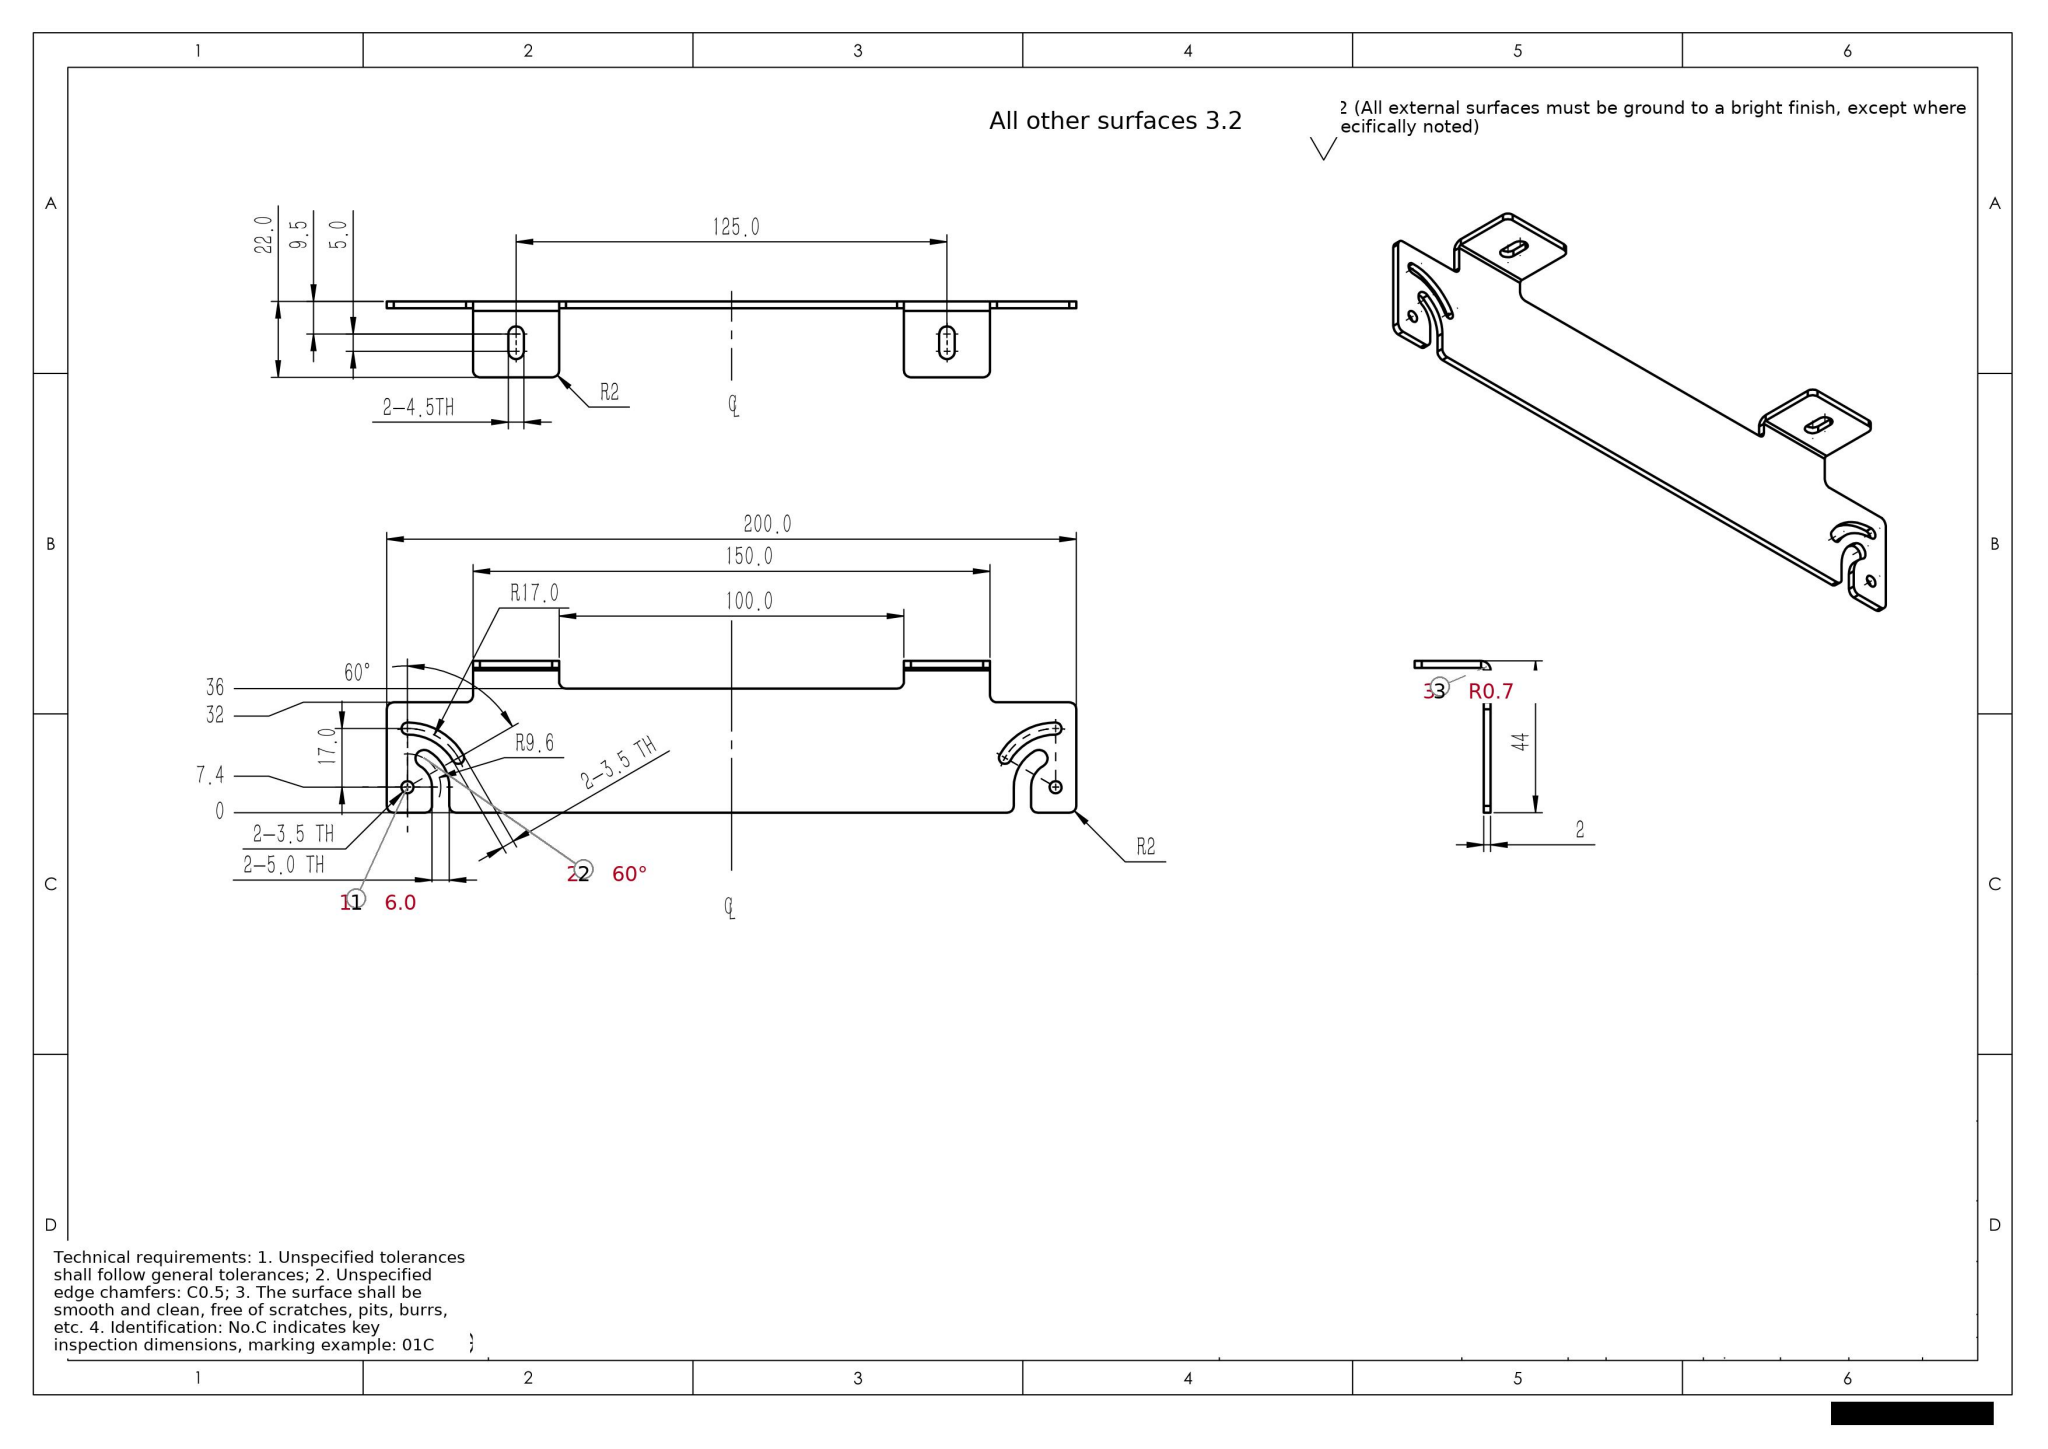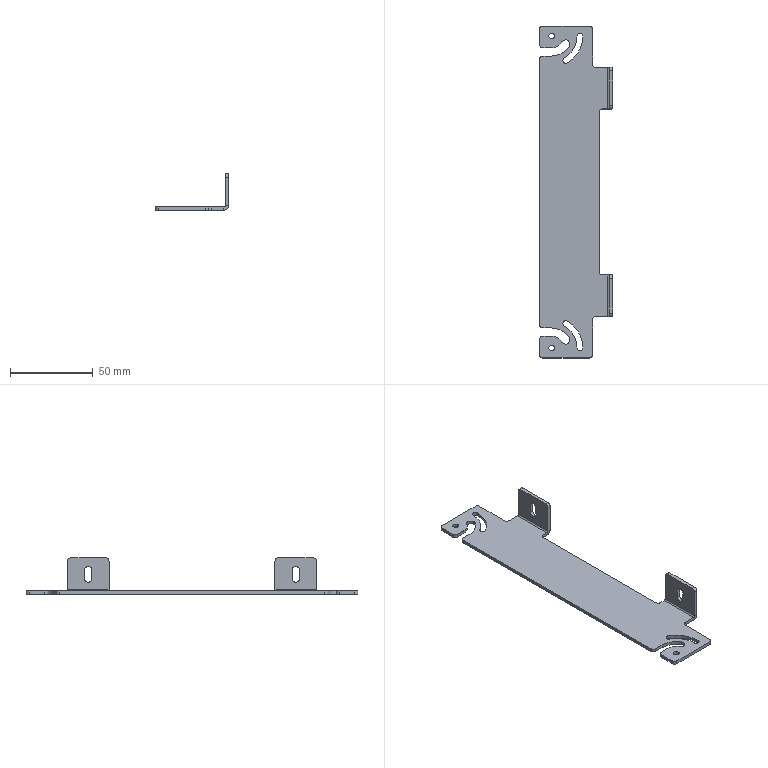Part | SolidWorks | mm | 1 solid | 82 faces | box 44 x 200 x 22 mm | volume 15843 mm3 | cylinder 46 | plane 36 | commonest cylinder face diameters 4 x16 3.5 x10 4.5 x6 5.473 x2 1.473 x2 24.24 x2 14.24 x2 5 x2